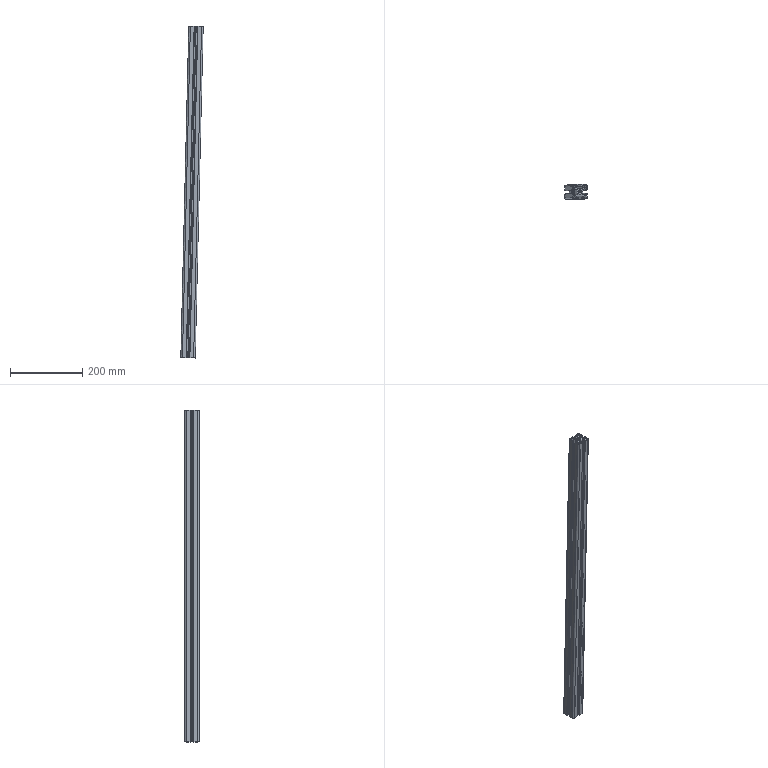Component | SolidWorks | 2012MB0201-1_AUpperRackFrameModule-1_A3008-3 | 1 solid | 201 faces | box 62 x 40 x 920.69 mm | volume 549306 mm3 | plane 151 | cylinder 50 | commonest cylinder face diameters 2 x12 19 x10 1 x8 6.8 x7 9 x4 5 x4 1.414 x3 6.6 x2
build123d program:
from build123d import *

# Parameters (mm, degrees)
BOSS_EXTRUDE1_DEPTH         = 920
SKETCH2_2_R                 = 9.5
CUT_EXTRUDE1_DEPTH          = 18
SKETCH1_R                   = 3.3
BOLT_CLEARANCE_HOLE_1_DEPTH = 11
BOLT_START                  = -11
SKETCH2_R                   = 3.3
BOLT_CLEARANCE_HOLE2_DEPTH  = 11


with BuildPart() as part:
    # Sketch1_2 → Boss-Extrude1 (new body)
    with BuildSketch(Plane.XY):
        with BuildLine():
            Line((-19, -4.1), (-19, -5.1))
            Line((-19, -5.1), (-20, -5.1))
            Line((-20, -5.1), (-20, -15.5))
            ThreePointArc((-20, -15.5), (-18.681, -18.682), (-15.499, -20))
            Line((-15.499, -20), (-5.099, -20))
            Line((-5.099, -20), (-5.099, -19))
            Line((-5.099, -19), (-4.099, -19))
            Line((-4.099, -19), (-4.099, -15.5))
            Line((-4.099, -15.5), (-6.599, -15.5))
            Line((-6.599, -15.5), (-6.599, -16.5))
            ThreePointArc((-6.599, -16.5), (-6.892, -17.207), (-7.599, -17.5))
            Line((-7.599, -17.5), (-9.8, -17.5))
            ThreePointArc((-9.8, -17.5), (-10.153, -17.354), (-10.3, -17))
            Line((-10.3, -17), (-10.3, -11.997))
            Line((-10.3, -11.997), (-5.902, -7.6))
            Line((-5.902, -7.6), (-0.5195, -7.6))
            Line((-0.5195, -7.6), (0.0005, -7.3))
            Line((0.0005, -7.3), (0.5195, -7.6))
            Line((0.5195, -7.6), (5.904, -7.6))
            Line((5.904, -7.6), (10.3, -11.997))
            Line((10.3, -11.997), (10.3, -17))
            ThreePointArc((10.3, -17), (10.154, -17.354), (9.8, -17.5))
            Line((9.8, -17.5), (7.601, -17.5))
            ThreePointArc((7.601, -17.5), (6.893, -17.207), (6.601, -16.5))
            Line((6.601, -16.5), (6.601, -15.5))
            Line((6.601, -15.5), (4.101, -15.5))
            Line((4.101, -15.5), (4.101, -19))
            Line((4.101, -19), (5.101, -19))
            Line((5.101, -19), (5.101, -20))
            Line((5.101, -20), (15.501, -20))
            ThreePointArc((15.501, -20), (18.682, -18.682), (20, -15.5))
            Line((20, -15.5), (20, -5.1))
            Line((20, -5.1), (19, -5.1))
            Line((19, -5.1), (19, -4.1))
            Line((19, -4.1), (15.501, -4.1))
            Line((15.501, -4.1), (15.501, -6.6))
            Line((15.501, -6.6), (16.5, -6.6))
            ThreePointArc((16.5, -6.6), (17.208, -6.893), (17.5, -7.6))
            Line((17.5, -7.6), (17.5, -9.8))
            ThreePointArc((17.5, -9.8), (17.354, -10.154), (17, -10.3))
            Line((17, -10.3), (11.998, -10.3))
            Line((11.998, -10.3), (7.601, -5.903))
            Line((7.601, -5.903), (7.601, -0.5203))
            Line((7.601, -0.5203), (7.301, -0.0003417))
            Line((7.301, -0.0003417), (7.601, 0.5197))
            Line((7.601, 0.5197), (7.601, 5.903))
            Line((7.601, 5.903), (11.998, 10.3))
            Line((11.998, 10.3), (17, 10.3))
            ThreePointArc((17, 10.3), (17.354, 10.153), (17.5, 9.8))
            Line((17.5, 9.8), (17.5, 7.6))
            ThreePointArc((17.5, 7.6), (17.208, 6.893), (16.5, 6.6))
            Line((16.5, 6.6), (15.501, 6.6))
            Line((15.501, 6.6), (15.501, 4.1))
            Line((15.501, 4.1), (19, 4.1))
            Line((19, 4.1), (19, 5.1))
            Line((19, 5.1), (20, 5.1))
            Line((20, 5.1), (20, 15.5))
            ThreePointArc((20, 15.5), (18.682, 18.682), (15.501, 20))
            Line((15.501, 20), (5.101, 20))
            Line((5.101, 20), (5.101, 19))
            Line((5.101, 19), (4.101, 19))
            Line((4.101, 19), (4.101, 15.5))
            Line((4.101, 15.5), (6.601, 15.5))
            ThreePointArc((6.601, 15.5), (6.393, 16), (6.601, 16.5))
            ThreePointArc((6.601, 16.5), (6.893, 17.207), (7.601, 17.5))
            Line((7.601, 17.5), (9.8, 17.5))
            ThreePointArc((9.8, 17.5), (10.154, 17.353), (10.3, 17))
            Line((10.3, 17), (10.3, 11.997))
            Line((10.3, 11.997), (5.904, 7.6))
            Line((5.904, 7.6), (0.5195, 7.6))
            Line((0.5195, 7.6), (0.0005, 7.3))
            Line((0.0005, 7.3), (-0.5195, 7.6))
            Line((-0.5195, 7.6), (-5.902, 7.6))
            Line((-5.902, 7.6), (-10.3, 11.997))
            Line((-10.3, 11.997), (-10.3, 17))
            ThreePointArc((-10.3, 17), (-10.153, 17.353), (-9.8, 17.5))
            Line((-9.8, 17.5), (-7.599, 17.5))
            ThreePointArc((-7.599, 17.5), (-6.892, 17.207), (-6.599, 16.5))
            Line((-6.599, 16.5), (-6.599, 15.5))
            Line((-6.599, 15.5), (-4.099, 15.5))
            Line((-4.099, 15.5), (-4.099, 19))
            Line((-4.099, 19), (-5.099, 19))
            Line((-5.099, 19), (-5.099, 20))
            Line((-5.099, 20), (-15.499, 20))
            ThreePointArc((-15.499, 20), (-18.681, 18.682), (-20, 15.5))
            Line((-20, 15.5), (-20, 5.1))
            Line((-20, 5.1), (-19, 5.1))
            Line((-19, 5.1), (-19, 4.1))
            Line((-19, 4.1), (-15.499, 4.1))
            Line((-15.499, 4.1), (-15.499, 6.6))
            Line((-15.499, 6.6), (-16.5, 6.6))
            ThreePointArc((-16.5, 6.6), (-17.207, 6.893), (-17.5, 7.6))
            Line((-17.5, 7.6), (-17.5, 9.8))
            ThreePointArc((-17.5, 9.8), (-17.353, 10.153), (-17, 10.3))
            Line((-17, 10.3), (-11.996, 10.3))
            Line((-11.996, 10.3), (-7.599, 5.903))
            Line((-7.599, 5.903), (-7.599, 0.5197))
            Line((-7.599, 0.5197), (-7.3, -0.0003417))
            Line((-7.3, -0.0003417), (-7.599, -0.5203))
            Line((-7.599, -0.5203), (-7.599, -5.903))
            Line((-7.599, -5.903), (-11.996, -10.3))
            Line((-11.996, -10.3), (-17, -10.3))
            ThreePointArc((-17, -10.3), (-17.353, -10.154), (-17.5, -9.8))
            Line((-17.5, -9.8), (-17.5, -7.6))
            ThreePointArc((-17.5, -7.6), (-17.207, -6.893), (-16.5, -6.6))
            Line((-16.5, -6.6), (-15.499, -6.6))
            Line((-15.499, -6.6), (-15.499, -4.1))
            Line((-15.499, -4.1), (-19, -4.1))
        make_face()
        with BuildLine():
            Line((15.501, -18), (11.8, -18))
            Line((11.8, -18), (11.8, -11.8))
            Line((11.8, -11.8), (18, -11.8))
            Line((18, -11.8), (18, -15.5))
            ThreePointArc((18, -15.5), (17.268, -17.268), (15.501, -18))
        make_face(mode=Mode.SUBTRACT)
        with BuildLine():
            Line((18, 11.8), (11.8, 11.8))
            Line((11.8, 11.8), (11.8, 18))
            Line((11.8, 18), (15.501, 18))
            ThreePointArc((15.501, 18), (17.268, 17.267), (18, 15.5))
            Line((18, 15.5), (18, 11.8))
        make_face(mode=Mode.SUBTRACT)
        with BuildLine():
            Line((-1.815, -2.875), (-3.004, -4.066))
            Line((-3.004, -4.066), (-4.066, -3.005))
            Line((-4.066, -3.005), (-2.874, -1.815))
            ThreePointArc((-2.874, -1.815), (-3.399, -0.0003417), (-2.874, 1.815))
            Line((-2.874, 1.815), (-4.064, 3.006))
            Line((-4.064, 3.006), (-3.004, 4.066))
            Line((-3.004, 4.066), (-1.815, 2.875))
            ThreePointArc((-1.815, 2.875), (0, 3.399), (1.815, 2.875))
            Line((1.815, 2.875), (3.006, 4.066))
            Line((3.006, 4.066), (4.067, 3.005))
            Line((4.067, 3.005), (2.876, 1.815))
            ThreePointArc((2.876, 1.815), (3.4, -0.0003417), (2.876, -1.815))
            Line((2.876, -1.815), (4.067, -3.005))
            Line((4.067, -3.005), (3.006, -4.066))
            Line((3.006, -4.066), (1.815, -2.875))
            ThreePointArc((1.815, -2.875), (0, -3.4), (-1.815, -2.875))
        make_face(mode=Mode.SUBTRACT)
        with BuildLine():
            Line((-18, -15.5), (-18, -11.8))
            Line((-18, -11.8), (-11.8, -11.8))
            Line((-11.8, -11.8), (-11.8, -18))
            Line((-11.8, -18), (-15.499, -18))
            ThreePointArc((-15.499, -18), (-17.267, -17.268), (-18, -15.5))
        make_face(mode=Mode.SUBTRACT)
        with BuildLine():
            Line((-11.8, 18), (-11.8, 11.8))
            Line((-11.8, 11.8), (-18, 11.8))
            Line((-18, 11.8), (-18, 15.5))
            ThreePointArc((-18, 15.5), (-17.267, 17.267), (-15.499, 18))
            Line((-15.499, 18), (-11.8, 18))
        make_face(mode=Mode.SUBTRACT)
    extrude(amount=-BOSS_EXTRUDE1_DEPTH)

    # Sketch2_2 → Cut-Extrude1 (cut)
    with BuildSketch(Plane(origin=(0, 20, 0), x_dir=(1, 0, 0), z_dir=(0, 1, 0))):
        with Locations(Location((0, 19, 0), (0, 0, 216.875))):
            Circle(SKETCH2_2_R)
        with Locations(Location((0, 901, 0), (0, 0, 216.875))):
            Circle(SKETCH2_2_R)
    extrude(amount=-CUT_EXTRUDE1_DEPTH, mode=Mode.SUBTRACT)

    # Sketch1 → Bolt Clearance Hole 1 (cut)
    with BuildSketch(Plane.XY):
        with Locations((0, 10)):
            Circle(SKETCH1_R)
    extrude(amount=-BOLT_CLEARANCE_HOLE_1_DEPTH, mode=Mode.SUBTRACT)

    # Sketch2 → Bolt Clearance Hole2 (cut)
    with BuildSketch(Plane(origin=(0, 0, -920), x_dir=(-1, 0, 0), z_dir=(0, 0, -1)).offset(BOLT_START)):
        with Locations((0, 10)):
            Circle(SKETCH2_R)
    extrude(amount=BOLT_CLEARANCE_HOLE2_DEPTH, mode=Mode.SUBTRACT)


solid = part.part

# Placed as in the assembly
solid = solid.moved(Location((-824.72, 1023.851, -1142.556), (-180, -1.371, -180)))